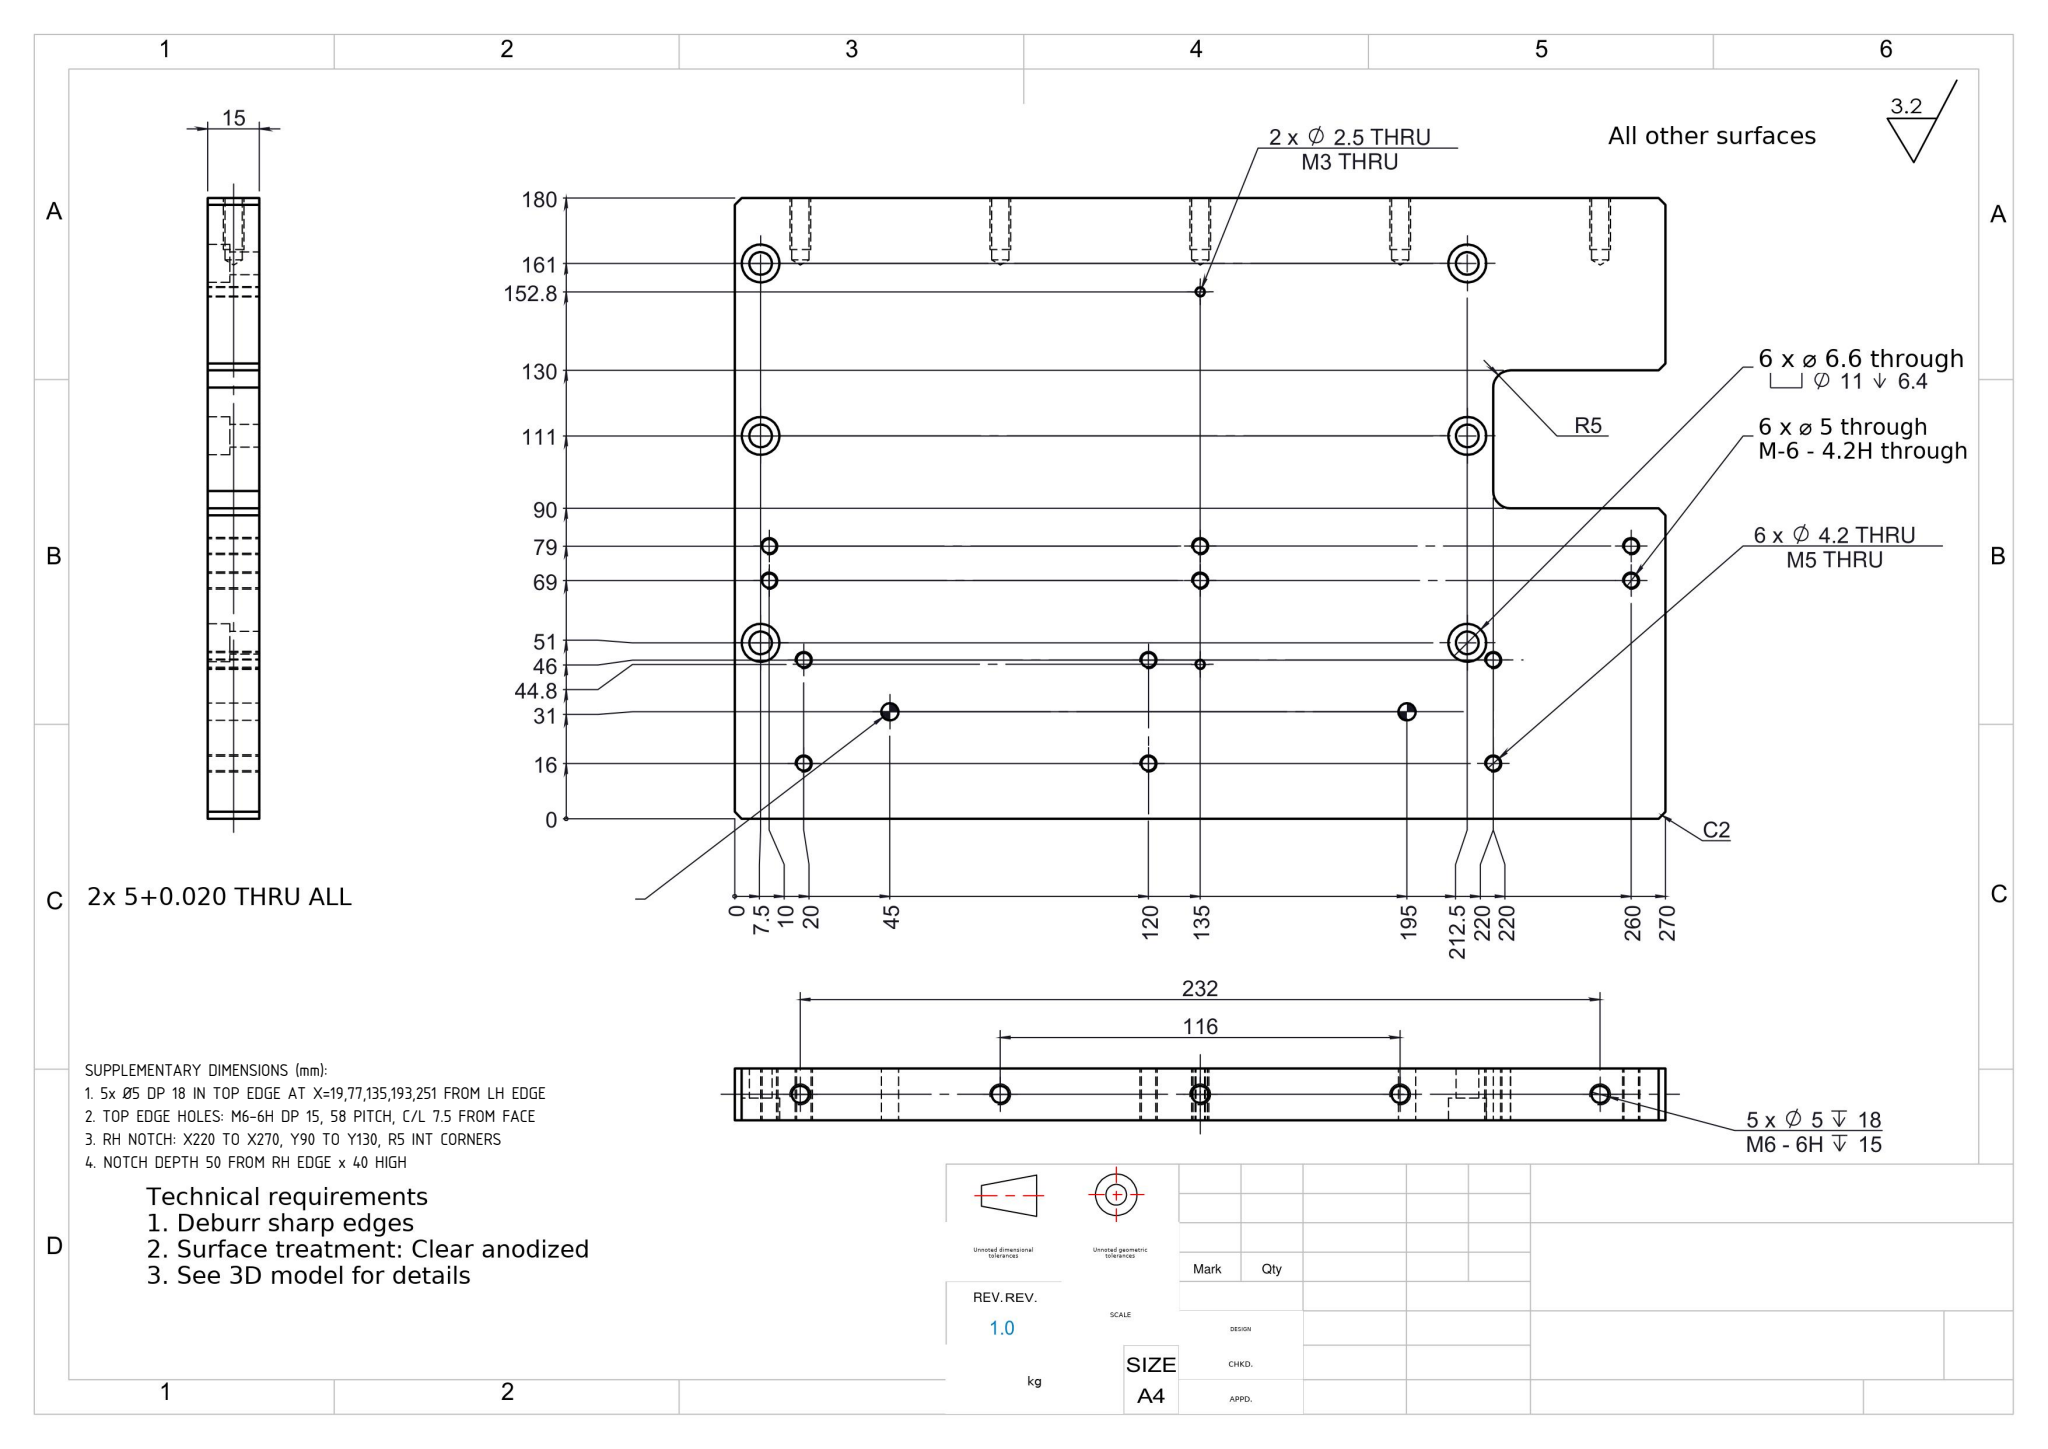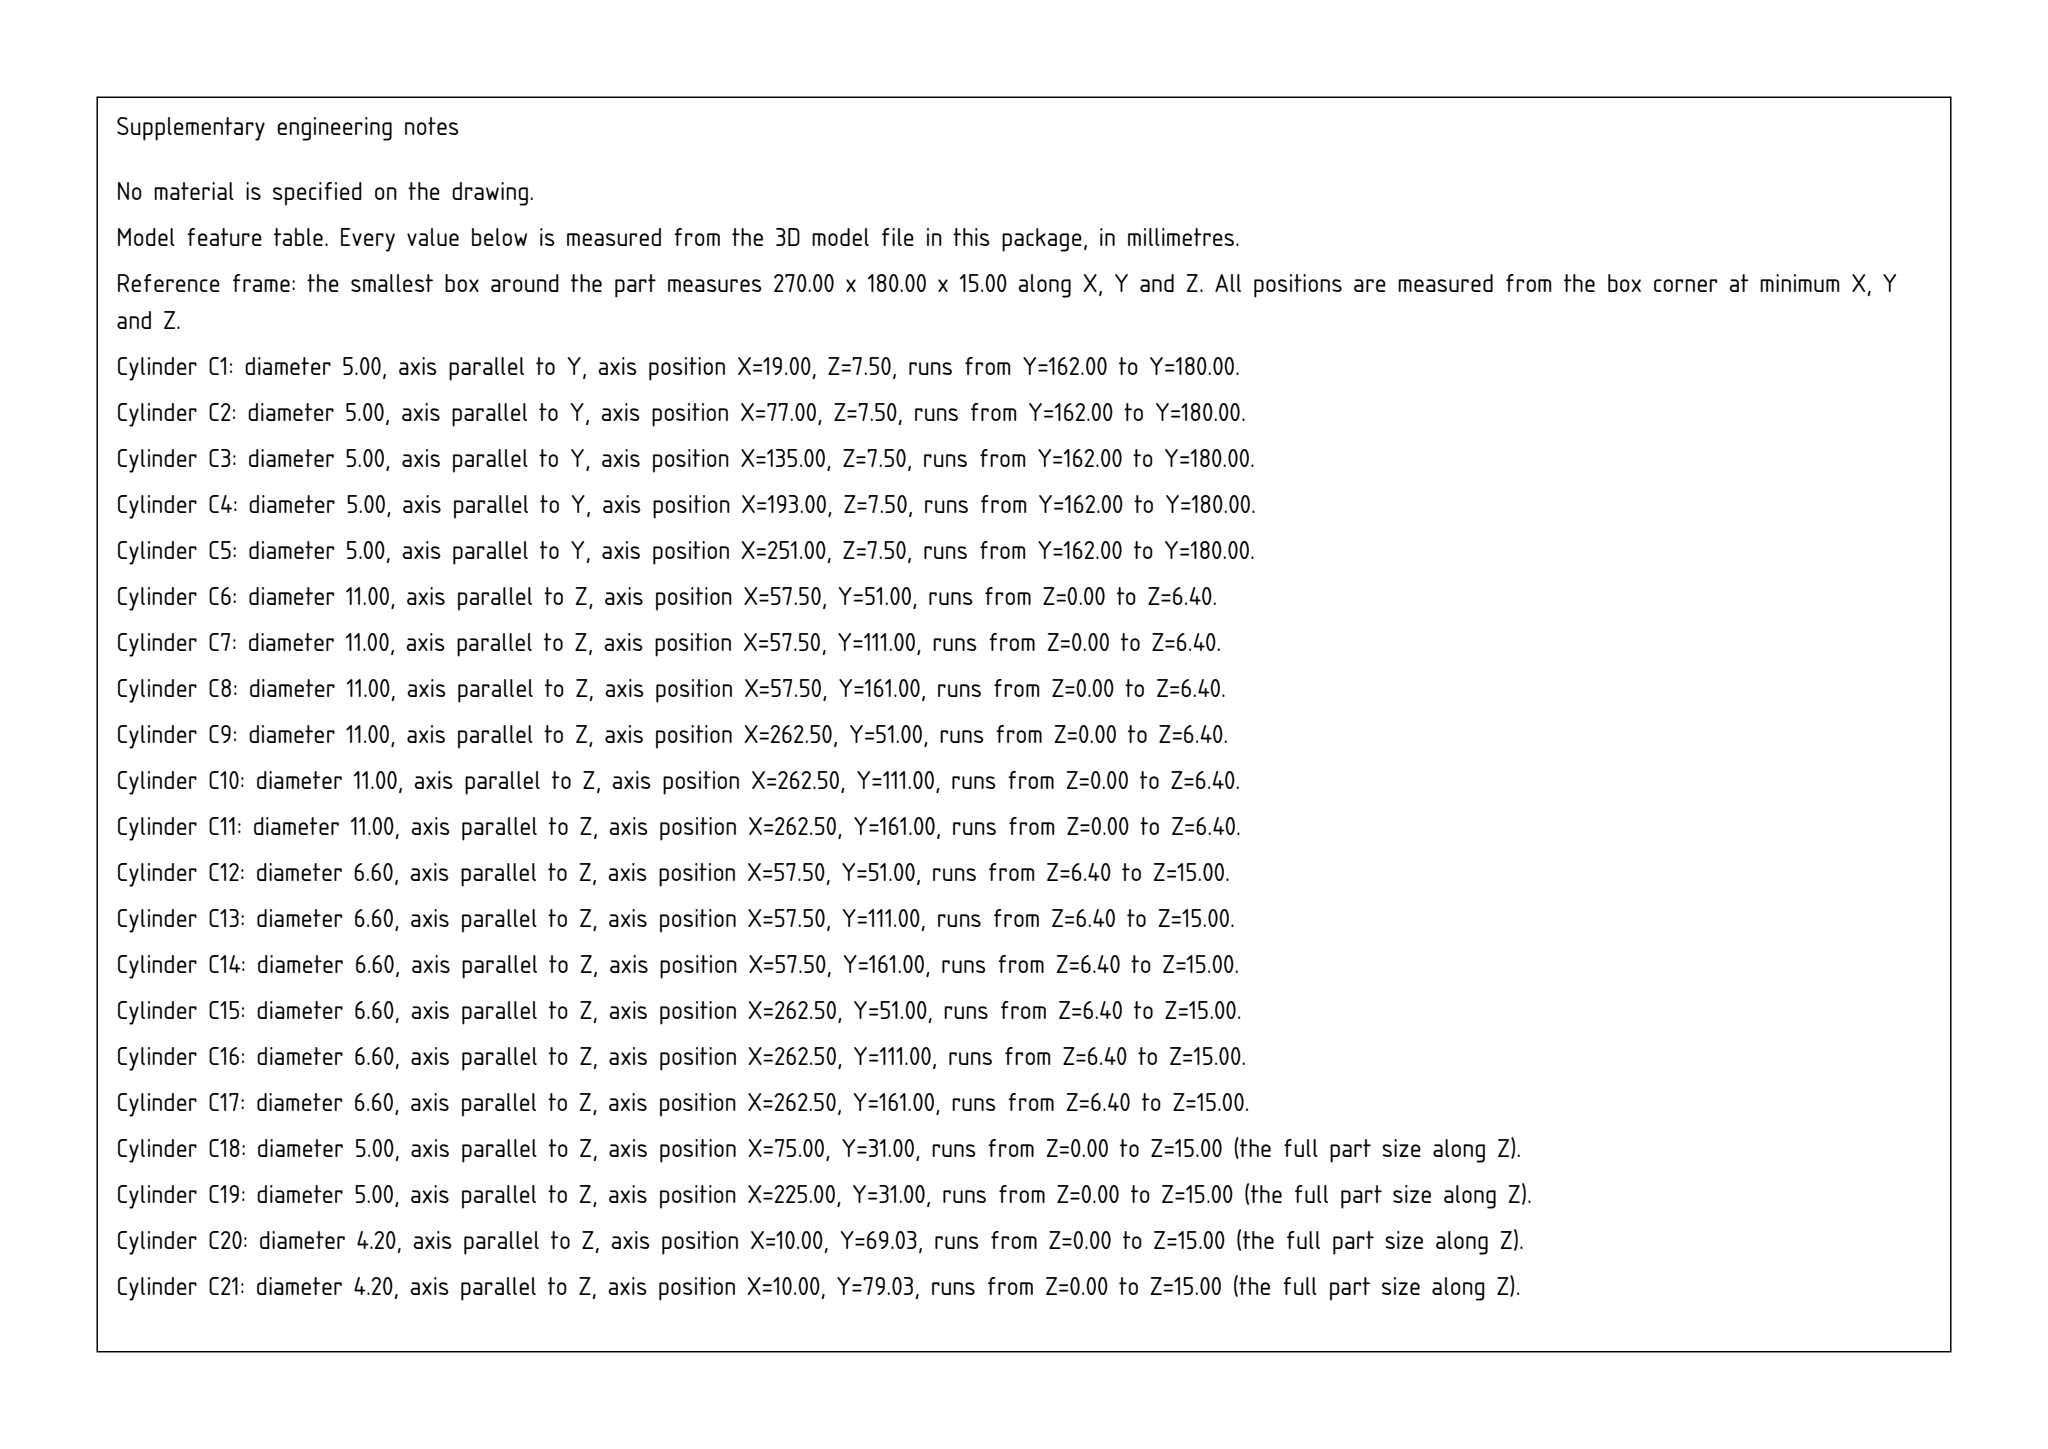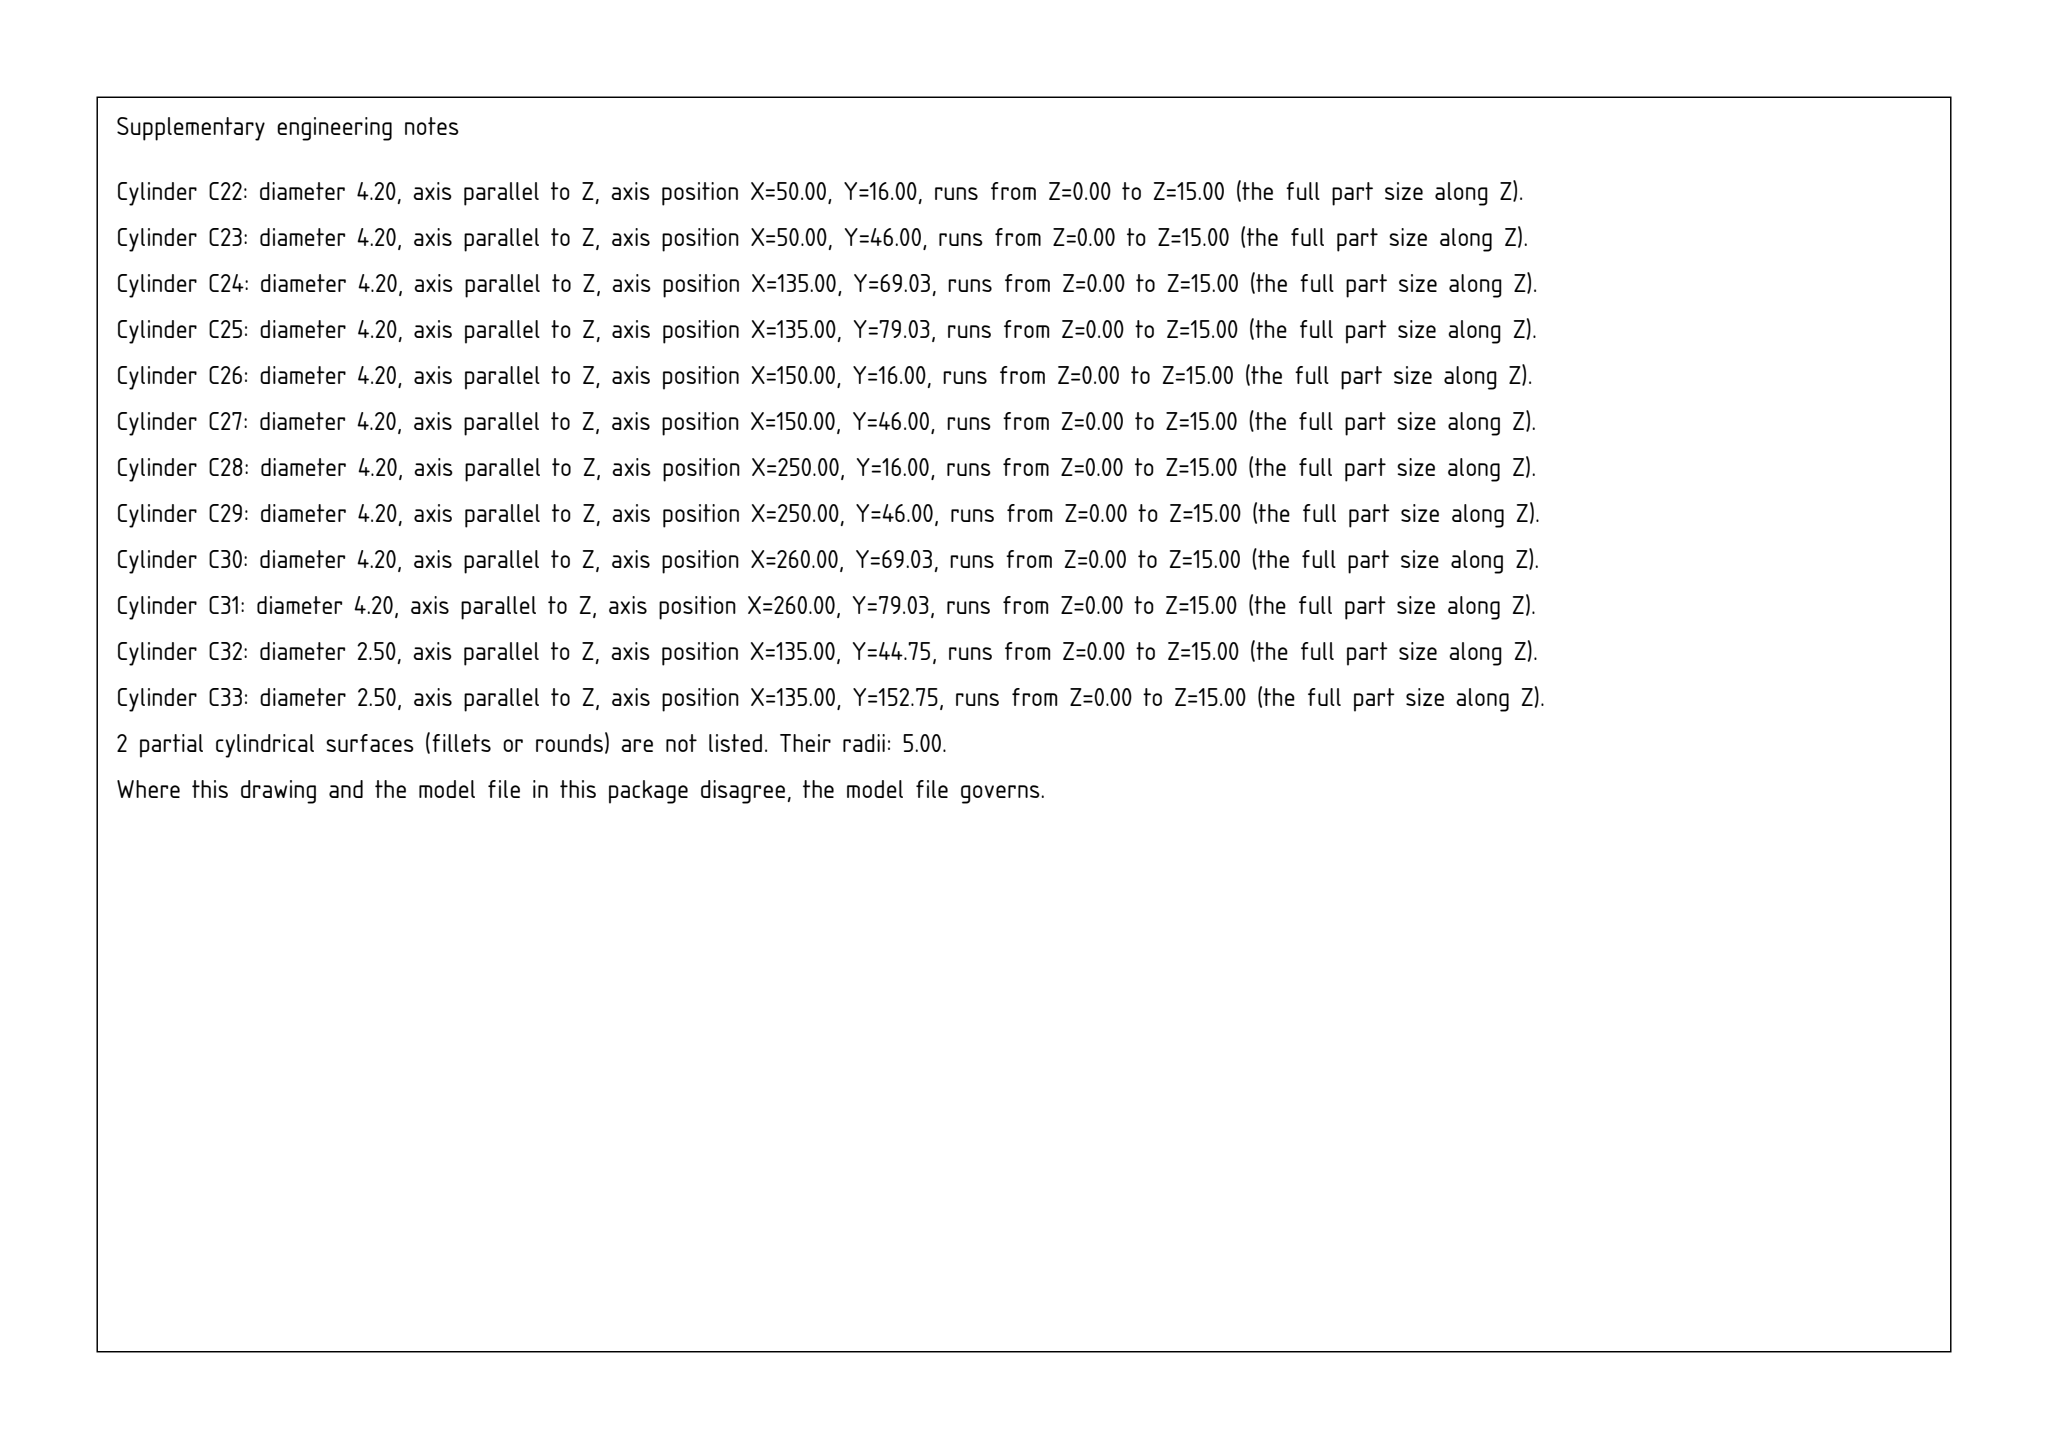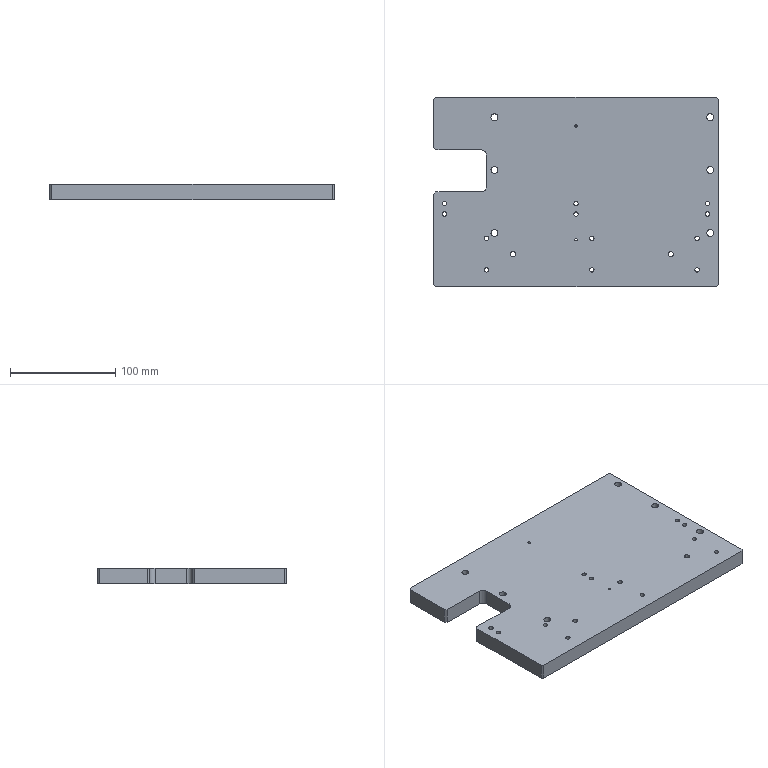Part | SolidWorks | mm | 1 solid | 100 faces | box 270 x 180 x 15 mm | volume 688520 mm3 | cylinder 68 | plane 22 | cone 10 | commonest cylinder face diameters 4.2 x24 5 x14 11 x12 6.6 x12 2.5 x4 10 x2
build123d program:
from build123d import *

# Parameters (mm, degrees)
SKETCH1_W                                       = 270
SKETCH1_H                                       = 180
BOSS_EXTRUDE1_DEPTH                             = 7.5
M6_HEX_SOCKET_HEAD_CAP_SCREW_CBORE1_D           = 6.6
M6_HEX_SOCKET_HEAD_CAP_SCREW_CBORE1_CBORE_D     = 11
M6_HEX_SOCKET_HEAD_CAP_SCREW_CBORE1_CBORE_DEPTH = 6.4
M5_TAPPED_HOLE1_D                               = 4.2
M5_TAPPED_HOLE3_D                               = 4.2
SKETCH10_W                                      = 50
SKETCH10_H                                      = 40
CUT_EXTRUDE1_DEPTH                              = 163.942
FILLET1_R                                       = 5
CHAMFER2_SIZE                                   = 2
M6_TAPPED_HOLE1_D                               = 5
M6_TAPPED_HOLE1_DEPTH                           = 18
M6_TAPPED_HOLE1_TIP                             = 1.502
SIZE_MM_DOWEL_PIN_HOLE1_D                       = 5
M3_TAPPED_HOLE1_D                               = 2.5


with BuildPart() as part:
    # Sketch1 → Boss-Extrude1 (new, symmetric)
    with BuildSketch(Plane.XY):
        Rectangle(SKETCH1_W, SKETCH1_H)
    extrude(amount=BOSS_EXTRUDE1_DEPTH, both=True)

    # M6 Hex Socket Head Cap Screw CBORE1 (through all)
    with Locations(Plane(origin=(0, 0, -7.5), x_dir=(-1, 0, 0), z_dir=(0, 0, -1))):
        with Locations((77.5, 71), (77.5, 21), (77.5, -39), (-127.5, -39), (-127.5, 21), (-127.5, 71)):
            CounterBoreHole(M6_HEX_SOCKET_HEAD_CAP_SCREW_CBORE1_D / 2, M6_HEX_SOCKET_HEAD_CAP_SCREW_CBORE1_CBORE_D / 2, M6_HEX_SOCKET_HEAD_CAP_SCREW_CBORE1_CBORE_DEPTH)

    # M5 Tapped Hole1 (through all)
    with Locations(Plane(origin=(0, 0, -7.5), x_dir=(-1, 0, 0), z_dir=(0, 0, -1))):
        with Locations((-115, -44), (-115, -74), (-15, -44), (-15, -74), (85, -44), (85, -74)):
            Hole(M5_TAPPED_HOLE1_D / 2)

    # M5 Tapped Hole3 (through all)
    with Locations(Plane(origin=(0, 0, -7.5), x_dir=(-1, 0, 0), z_dir=(0, 0, -1))):
        with Locations((-125, -10.967), (-125, -20.967), (0, -10.967), (0, -20.967), (125, -10.967), (125, -20.967)):
            Hole(M5_TAPPED_HOLE3_D / 2)

    # Sketch10 → Cut-Extrude1 (cut, through all)
    with BuildSketch(Plane(origin=(0, 0, -7.5), x_dir=(-1, 0, 0), z_dir=(0, 0, -1))):
        with Locations((110, 20)):
            Rectangle(SKETCH10_W, SKETCH10_H)
    extrude(amount=-CUT_EXTRUDE1_DEPTH, mode=Mode.SUBTRACT)

    # Fillet1
    fillet1_edges = [part.edges().sort_by_distance(p)[0] for p in [
        (-85, 0, 0),
        (-85, 40, 0),
    ]]
    fillet(fillet1_edges, radius=FILLET1_R)

    # Chamfer2
    chamfer2_edges = [part.edges().sort_by_distance(p)[0] for p in [
        (-135, 40, 0),
        (-135, 0, 0),
        (-135, 90, 0),
        (135, 90, 0),
        (135, -90, 0),
        (-135, -90, 0),
    ]]
    chamfer(chamfer2_edges, length=CHAMFER2_SIZE)

    # M6 Tapped Hole1
    with Locations(Plane(origin=(0, 90, 0), x_dir=(1, 0, 0), z_dir=(0, 1, 0))):
        with Locations((-116, 0), (116, 0), (-58, 0), (58, 0), (0, 0)):
            Hole(M6_TAPPED_HOLE1_D / 2, depth=M6_TAPPED_HOLE1_DEPTH)
            with Locations((0, 0, -(M6_TAPPED_HOLE1_DEPTH + M6_TAPPED_HOLE1_TIP / 2))):  # 118° drill point
                Cone(0, M6_TAPPED_HOLE1_D / 2, M6_TAPPED_HOLE1_TIP, mode=Mode.SUBTRACT)

    # Size mm Dowel Pin Hole1 (through all)
    with Locations(Plane(origin=(0, 0, -7.5), x_dir=(-1, 0, 0), z_dir=(0, 0, -1))):
        with Locations((-90, -59), (60, -59)):
            Hole(SIZE_MM_DOWEL_PIN_HOLE1_D / 2)

    # M3 Tapped Hole1 (through all)
    with Locations(Plane.XY.offset(7.5)):
        with Locations((0, 62.75), (0, -45.25)):
            Hole(M3_TAPPED_HOLE1_D / 2)


solid = part.part